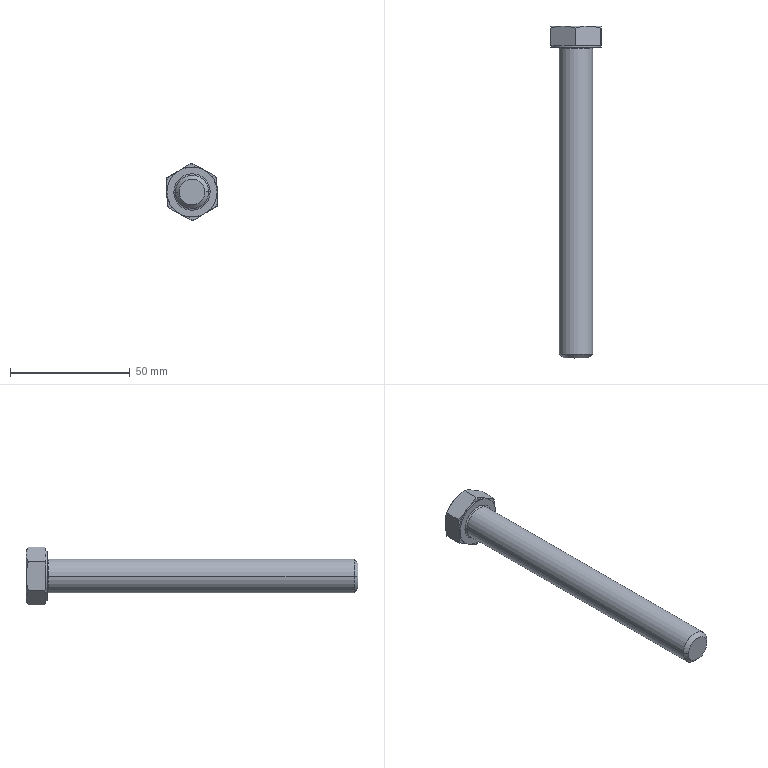Component | SolidWorks | 23HexHeadBolt_GradeAAndB[GBT5782-2000][M14_130_40]-4 | 1 solid | 35 faces | box 21.22 x 138.8 x 24.24 mm | volume 23292 mm3 | plane 15 | cone 14 | cylinder 4 | torus 2 | commonest cylinder face diameters 14 x2 21 x2 | material Steel
STEP:
#1=CARTESIAN_POINT('',(4.247,7.528,24.011));
#2=VERTEX_POINT('',#1);
#3=CARTESIAN_POINT('',(4.799,7.528,24.021));
#4=VERTEX_POINT('',#3);
#5=CARTESIAN_POINT('',(4.523,7.528,24.016));
#6=DIRECTION('',(0.,-1.,0.));
#7=DIRECTION('',(0.9998,0.,0.01816));
#8=AXIS2_PLACEMENT_3D('',#5,#6,#7);
#9=CIRCLE('',#8,0.2756);
#10=EDGE_CURVE('',#2,#4,#9,.T.);
#11=ORIENTED_EDGE('',*,*,#10,.F.);
#12=CARTESIAN_POINT('',(4.224,7.552,24.01));
#13=VERTEX_POINT('',#12);
#14=CARTESIAN_POINT('',(4.224,7.528,24.01));
#15=DIRECTION('',(-0.01816,0.,0.9998));
#16=DIRECTION('',(0.9998,0.,0.01816));
#17=AXIS2_PLACEMENT_3D('',#14,#15,#16);
#18=CIRCLE('',#17,0.02362);
#19=EDGE_CURVE('',#2,#13,#18,.T.);
#20=ORIENTED_EDGE('',*,*,#19,.T.);
#21=CARTESIAN_POINT('',(4.822,7.552,24.021));
#22=VERTEX_POINT('',#21);
#23=CARTESIAN_POINT('',(4.523,7.552,24.016));
#24=DIRECTION('',(0.,1.,0.));
#25=DIRECTION('',(0.9998,0.,0.01816));
#26=AXIS2_PLACEMENT_3D('',#23,#24,#25);
#27=CIRCLE('',#26,0.2992);
#28=EDGE_CURVE('',#22,#13,#27,.T.);
#29=ORIENTED_EDGE('',*,*,#28,.F.);
#30=CARTESIAN_POINT('',(4.822,7.528,24.021));
#31=DIRECTION('',(0.01816,0.,-0.9998));
#32=DIRECTION('',(-0.9998,0.,-0.01816));
#33=AXIS2_PLACEMENT_3D('',#30,#31,#32);
#34=CIRCLE('',#33,0.02362);
#35=EDGE_CURVE('',#4,#22,#34,.T.);
#36=ORIENTED_EDGE('',*,*,#35,.F.);
#37=EDGE_LOOP('',(#11,#20,#29,#36));
#38=FACE_OUTER_BOUND('',#37,.T.);
#39=CARTESIAN_POINT('',(4.523,7.528,24.016));
#40=DIRECTION('',(0.,-1.,0.));
#41=DIRECTION('',(0.9998,0.,0.01816));
#42=AXIS2_PLACEMENT_3D('',#39,#40,#41);
#43=TOROIDAL_SURFACE('',#42,0.2992,0.02362);
#44=ADVANCED_FACE('',(#38),#43,.F.);
#45=CARTESIAN_POINT('',(4.736,2.433,24.02));
#46=VERTEX_POINT('',#45);
#47=CARTESIAN_POINT('',(4.31,2.433,24.012));
#48=VERTEX_POINT('',#47);
#49=CARTESIAN_POINT('',(4.523,2.433,24.016));
#50=DIRECTION('',(0.,-1.,0.));
#51=DIRECTION('',(-0.9998,0.,-0.01816));
#52=AXIS2_PLACEMENT_3D('',#49,#50,#51);
#53=CIRCLE('',#52,0.2126);
#54=EDGE_CURVE('',#46,#48,#53,.T.);
#55=ORIENTED_EDGE('',*,*,#54,.F.);
#56=CARTESIAN_POINT('',(4.799,2.496,24.021));
#57=VERTEX_POINT('',#56);
#58=CARTESIAN_POINT('',(4.799,2.496,24.021));
#59=DIRECTION('',(0.707,0.7071,0.01284));
#60=VECTOR('',#59,39.37);
#61=LINE('',#58,#60);
#62=EDGE_CURVE('',#46,#57,#61,.T.);
#63=ORIENTED_EDGE('',*,*,#62,.T.);
#64=CARTESIAN_POINT('',(4.247,2.496,24.011));
#65=VERTEX_POINT('',#64);
#66=CARTESIAN_POINT('',(4.523,2.496,24.016));
#67=DIRECTION('',(0.,1.,0.));
#68=DIRECTION('',(-0.9998,0.,-0.01816));
#69=AXIS2_PLACEMENT_3D('',#66,#67,#68);
#70=CIRCLE('',#69,0.2756);
#71=EDGE_CURVE('',#65,#57,#70,.T.);
#72=ORIENTED_EDGE('',*,*,#71,.F.);
#73=CARTESIAN_POINT('',(4.247,2.496,24.011));
#74=DIRECTION('',(-0.707,0.7071,-0.01284));
#75=VECTOR('',#74,39.37);
#76=LINE('',#73,#75);
#77=EDGE_CURVE('',#48,#65,#76,.T.);
#78=ORIENTED_EDGE('',*,*,#77,.F.);
#79=EDGE_LOOP('',(#55,#63,#72,#78));
#80=FACE_OUTER_BOUND('',#79,.T.);
#81=CARTESIAN_POINT('',(4.523,2.496,24.016));
#82=DIRECTION('',(0.,1.,0.));
#83=DIRECTION('',(-0.9998,0.,-0.01816));
#84=AXIS2_PLACEMENT_3D('',#81,#82,#83);
#85=CONICAL_SURFACE('',#84,0.2756,0.7854);
#86=ADVANCED_FACE('',(#80),#85,.T.);
#87=ORIENTED_EDGE('',*,*,#71,.T.);
#88=CARTESIAN_POINT('',(4.799,7.898,24.021));
#89=DIRECTION('',(0.,1.,0.));
#90=VECTOR('',#89,39.37);
#91=LINE('',#88,#90);
#92=EDGE_CURVE('',#57,#4,#91,.T.);
#93=ORIENTED_EDGE('',*,*,#92,.T.);
#94=CARTESIAN_POINT('',(4.523,7.528,24.016));
#95=DIRECTION('',(0.,-1.,0.));
#96=DIRECTION('',(0.9998,0.,0.01816));
#97=AXIS2_PLACEMENT_3D('',#94,#95,#96);
#98=CIRCLE('',#97,0.2756);
#99=EDGE_CURVE('',#4,#2,#98,.T.);
#100=ORIENTED_EDGE('',*,*,#99,.T.);
#101=CARTESIAN_POINT('',(4.247,7.898,24.011));
#102=DIRECTION('',(0.,1.,0.));
#103=VECTOR('',#102,39.37);
#104=LINE('',#101,#103);
#105=EDGE_CURVE('',#65,#2,#104,.T.);
#106=ORIENTED_EDGE('',*,*,#105,.F.);
#107=EDGE_LOOP('',(#87,#93,#100,#106));
#108=FACE_OUTER_BOUND('',#107,.T.);
#109=CARTESIAN_POINT('',(4.523,7.898,24.016));
#110=DIRECTION('',(0.,1.,0.));
#111=DIRECTION('',(-0.9998,0.,-0.01816));
#112=AXIS2_PLACEMENT_3D('',#109,#110,#111);
#113=CYLINDRICAL_SURFACE('',#112,0.2756);
#114=ADVANCED_FACE('',(#108),#113,.T.);
#115=CARTESIAN_POINT('',(4.936,7.552,24.023));
#116=VERTEX_POINT('',#115);
#117=CARTESIAN_POINT('',(4.11,7.552,24.008));
#118=VERTEX_POINT('',#117);
#119=CARTESIAN_POINT('',(4.523,7.552,24.016));
#120=DIRECTION('',(0.,-1.,0.));
#121=DIRECTION('',(0.9998,0.,0.01816));
#122=AXIS2_PLACEMENT_3D('',#119,#120,#121);
#123=CIRCLE('',#122,0.4134);
#124=EDGE_CURVE('',#116,#118,#123,.T.);
#125=ORIENTED_EDGE('',*,*,#124,.F.);
#126=CARTESIAN_POINT('',(4.936,7.575,24.023));
#127=VERTEX_POINT('',#126);
#128=CARTESIAN_POINT('',(4.936,7.898,24.023));
#129=DIRECTION('',(0.,1.,0.));
#130=VECTOR('',#129,39.37);
#131=LINE('',#128,#130);
#132=EDGE_CURVE('',#116,#127,#131,.T.);
#133=ORIENTED_EDGE('',*,*,#132,.T.);
#134=CARTESIAN_POINT('',(4.723,7.575,24.377));
#135=VERTEX_POINT('',#134);
#136=CARTESIAN_POINT('',(4.523,7.575,24.016));
#137=DIRECTION('',(0.,1.,0.));
#138=DIRECTION('',(-0.9998,0.,-0.01816));
#139=AXIS2_PLACEMENT_3D('',#136,#137,#138);
#140=CIRCLE('',#139,0.4134);
#141=EDGE_CURVE('',#135,#127,#140,.T.);
#142=ORIENTED_EDGE('',*,*,#141,.F.);
#143=CARTESIAN_POINT('',(4.31,7.575,24.37));
#144=VERTEX_POINT('',#143);
#145=CARTESIAN_POINT('',(4.523,7.575,24.016));
#146=DIRECTION('',(0.,1.,0.));
#147=DIRECTION('',(-0.9998,0.,-0.01816));
#148=AXIS2_PLACEMENT_3D('',#145,#146,#147);
#149=CIRCLE('',#148,0.4134);
#150=EDGE_CURVE('',#144,#135,#149,.T.);
#151=ORIENTED_EDGE('',*,*,#150,.F.);
#152=CARTESIAN_POINT('',(4.11,7.575,24.008));
#153=VERTEX_POINT('',#152);
#154=CARTESIAN_POINT('',(4.523,7.575,24.016));
#155=DIRECTION('',(0.,1.,0.));
#156=DIRECTION('',(-0.9998,0.,-0.01816));
#157=AXIS2_PLACEMENT_3D('',#154,#155,#156);
#158=CIRCLE('',#157,0.4134);
#159=EDGE_CURVE('',#153,#144,#158,.T.);
#160=ORIENTED_EDGE('',*,*,#159,.F.);
#161=CARTESIAN_POINT('',(4.11,7.898,24.008));
#162=DIRECTION('',(0.,1.,0.));
#163=VECTOR('',#162,39.37);
#164=LINE('',#161,#163);
#165=EDGE_CURVE('',#118,#153,#164,.T.);
#166=ORIENTED_EDGE('',*,*,#165,.F.);
#167=EDGE_LOOP('',(#125,#133,#142,#151,#160,#166));
#168=FACE_OUTER_BOUND('',#167,.T.);
#169=CARTESIAN_POINT('',(4.523,7.898,24.016));
#170=DIRECTION('',(0.,1.,0.));
#171=DIRECTION('',(-0.9998,0.,-0.01816));
#172=AXIS2_PLACEMENT_3D('',#169,#170,#171);
#173=CYLINDRICAL_SURFACE('',#172,0.4134);
#174=ADVANCED_FACE('',(#168),#173,.T.);
#175=CARTESIAN_POINT('',(4.888,7.575,24.286));
#176=VERTEX_POINT('',#175);
#177=CARTESIAN_POINT('',(4.932,7.575,24.262));
#178=DIRECTION('',(-0.875,0.,0.4842));
#179=VECTOR('',#178,39.37);
#180=LINE('',#177,#179);
#181=EDGE_CURVE('',#176,#135,#180,.T.);
#182=ORIENTED_EDGE('',*,*,#181,.F.);
#183=CARTESIAN_POINT('',(4.932,7.588,24.262));
#184=VERTEX_POINT('',#183);
#185=CARTESIAN_POINT('',(4.932,7.588,24.262));
#186=CARTESIAN_POINT('',(4.917,7.584,24.27));
#187=CARTESIAN_POINT('',(4.903,7.579,24.278));
#188=CARTESIAN_POINT('',(4.888,7.575,24.286));
#189=B_SPLINE_CURVE_WITH_KNOTS('',3,(#185,#186,#187,#188),.UNSPECIFIED.,.F.,.F.,(4,4),(0.00000024,0.001312),.UNSPECIFIED.);
#190=EDGE_CURVE('',#184,#176,#189,.T.);
#191=ORIENTED_EDGE('',*,*,#190,.F.);
#192=CARTESIAN_POINT('',(4.932,7.861,24.262));
#193=VERTEX_POINT('',#192);
#194=CARTESIAN_POINT('',(4.932,7.552,24.262));
#195=DIRECTION('',(0.,1.,0.));
#196=VECTOR('',#195,39.37);
#197=LINE('',#194,#196);
#198=EDGE_CURVE('',#184,#193,#197,.T.);
#199=ORIENTED_EDGE('',*,*,#198,.T.);
#200=CARTESIAN_POINT('',(4.723,7.898,24.377));
#201=VERTEX_POINT('',#200);
#202=CARTESIAN_POINT('',(4.723,7.898,24.377));
#203=CARTESIAN_POINT('',(4.741,7.898,24.368));
#204=CARTESIAN_POINT('',(4.759,7.897,24.358));
#205=CARTESIAN_POINT('',(4.794,7.894,24.338));
#206=CARTESIAN_POINT('',(4.811,7.891,24.329));
#207=CARTESIAN_POINT('',(4.864,7.882,24.3));
#208=CARTESIAN_POINT('',(4.898,7.872,24.281));
#209=CARTESIAN_POINT('',(4.932,7.861,24.262));
#210=B_SPLINE_CURVE_WITH_KNOTS('',3,(#202,#203,#204,#205,#206,#207,#208,#209),.UNSPECIFIED.,.F.,.F.,(4,2,2,4),(0.006134,0.007662,0.00919,0.01225),.UNSPECIFIED.);
#211=EDGE_CURVE('',#201,#193,#210,.T.);
#212=ORIENTED_EDGE('',*,*,#211,.F.);
#213=CARTESIAN_POINT('',(4.514,7.861,24.493));
#214=VERTEX_POINT('',#213);
#215=CARTESIAN_POINT('',(4.514,7.861,24.493));
#216=CARTESIAN_POINT('',(4.549,7.872,24.474));
#217=CARTESIAN_POINT('',(4.583,7.882,24.455));
#218=CARTESIAN_POINT('',(4.652,7.894,24.417));
#219=CARTESIAN_POINT('',(4.688,7.898,24.397));
#220=CARTESIAN_POINT('',(4.723,7.898,24.377));
#221=B_SPLINE_CURVE_WITH_KNOTS('',3,(#215,#216,#217,#218,#219,#220),.UNSPECIFIED.,.F.,.F.,(4,2,4),(0.00000024,0.003067,0.006134),.UNSPECIFIED.);
#222=EDGE_CURVE('',#214,#201,#221,.T.);
#223=ORIENTED_EDGE('',*,*,#222,.F.);
#224=CARTESIAN_POINT('',(4.514,7.588,24.493));
#225=VERTEX_POINT('',#224);
#226=CARTESIAN_POINT('',(4.514,7.552,24.493));
#227=DIRECTION('',(0.,1.,0.));
#228=VECTOR('',#227,39.37);
#229=LINE('',#226,#228);
#230=EDGE_CURVE('',#225,#214,#229,.T.);
#231=ORIENTED_EDGE('',*,*,#230,.F.);
#232=CARTESIAN_POINT('',(4.558,7.575,24.469));
#233=VERTEX_POINT('',#232);
#234=CARTESIAN_POINT('',(4.558,7.575,24.469));
#235=CARTESIAN_POINT('',(4.544,7.579,24.477));
#236=CARTESIAN_POINT('',(4.529,7.584,24.485));
#237=CARTESIAN_POINT('',(4.514,7.588,24.493));
#238=B_SPLINE_CURVE_WITH_KNOTS('',3,(#234,#235,#236,#237),.UNSPECIFIED.,.F.,.F.,(4,4),(0.01094,0.01225),.UNSPECIFIED.);
#239=EDGE_CURVE('',#233,#225,#238,.T.);
#240=ORIENTED_EDGE('',*,*,#239,.F.);
#241=CARTESIAN_POINT('',(4.932,7.575,24.262));
#242=DIRECTION('',(-0.875,0.,0.4842));
#243=VECTOR('',#242,39.37);
#244=LINE('',#241,#243);
#245=EDGE_CURVE('',#135,#233,#244,.T.);
#246=ORIENTED_EDGE('',*,*,#245,.F.);
#247=EDGE_LOOP('',(#182,#191,#199,#212,#223,#231,#240,#246));
#248=FACE_OUTER_BOUND('',#247,.T.);
#249=CARTESIAN_POINT('',(4.932,7.552,24.262));
#250=DIRECTION('',(-0.4842,0.,-0.875));
#251=DIRECTION('',(0.875,0.,-0.4842));
#252=AXIS2_PLACEMENT_3D('',#249,#250,#251);
#253=PLANE('',#252);
#254=ADVANCED_FACE('',(#248),#253,.F.);
#255=CARTESIAN_POINT('',(4.471,7.575,24.467));
#256=VERTEX_POINT('',#255);
#257=CARTESIAN_POINT('',(4.514,7.575,24.493));
#258=DIRECTION('',(-0.8568,0.,-0.5156));
#259=VECTOR('',#258,39.37);
#260=LINE('',#257,#259);
#261=EDGE_CURVE('',#256,#144,#260,.T.);
#262=ORIENTED_EDGE('',*,*,#261,.F.);
#263=CARTESIAN_POINT('',(4.514,7.588,24.493));
#264=CARTESIAN_POINT('',(4.5,7.584,24.484));
#265=CARTESIAN_POINT('',(4.486,7.579,24.476));
#266=CARTESIAN_POINT('',(4.471,7.575,24.467));
#267=B_SPLINE_CURVE_WITH_KNOTS('',3,(#263,#264,#265,#266),.UNSPECIFIED.,.F.,.F.,(4,4),(0.00000024,0.001312),.UNSPECIFIED.);
#268=EDGE_CURVE('',#225,#256,#267,.T.);
#269=ORIENTED_EDGE('',*,*,#268,.F.);
#270=ORIENTED_EDGE('',*,*,#230,.T.);
#271=CARTESIAN_POINT('',(4.31,7.898,24.37));
#272=VERTEX_POINT('',#271);
#273=CARTESIAN_POINT('',(4.31,7.898,24.37));
#274=CARTESIAN_POINT('',(4.327,7.898,24.38));
#275=CARTESIAN_POINT('',(4.345,7.897,24.391));
#276=CARTESIAN_POINT('',(4.379,7.894,24.412));
#277=CARTESIAN_POINT('',(4.396,7.891,24.422));
#278=CARTESIAN_POINT('',(4.447,7.882,24.453));
#279=CARTESIAN_POINT('',(4.481,7.872,24.473));
#280=CARTESIAN_POINT('',(4.514,7.861,24.493));
#281=B_SPLINE_CURVE_WITH_KNOTS('',3,(#273,#274,#275,#276,#277,#278,#279,#280),.UNSPECIFIED.,.F.,.F.,(4,2,2,4),(0.006134,0.007662,0.00919,0.01225),.UNSPECIFIED.);
#282=EDGE_CURVE('',#272,#214,#281,.T.);
#283=ORIENTED_EDGE('',*,*,#282,.F.);
#284=CARTESIAN_POINT('',(4.105,7.861,24.247));
#285=VERTEX_POINT('',#284);
#286=CARTESIAN_POINT('',(4.105,7.861,24.247));
#287=CARTESIAN_POINT('',(4.139,7.872,24.267));
#288=CARTESIAN_POINT('',(4.173,7.882,24.287));
#289=CARTESIAN_POINT('',(4.241,7.894,24.328));
#290=CARTESIAN_POINT('',(4.275,7.898,24.349));
#291=CARTESIAN_POINT('',(4.31,7.898,24.37));
#292=B_SPLINE_CURVE_WITH_KNOTS('',3,(#286,#287,#288,#289,#290,#291),.UNSPECIFIED.,.F.,.F.,(4,2,4),(0.00000024,0.003067,0.006134),.UNSPECIFIED.);
#293=EDGE_CURVE('',#285,#272,#292,.T.);
#294=ORIENTED_EDGE('',*,*,#293,.F.);
#295=CARTESIAN_POINT('',(4.105,7.588,24.247));
#296=VERTEX_POINT('',#295);
#297=CARTESIAN_POINT('',(4.105,7.552,24.247));
#298=DIRECTION('',(0.,1.,0.));
#299=VECTOR('',#298,39.37);
#300=LINE('',#297,#299);
#301=EDGE_CURVE('',#296,#285,#300,.T.);
#302=ORIENTED_EDGE('',*,*,#301,.F.);
#303=CARTESIAN_POINT('',(4.148,7.575,24.273));
#304=VERTEX_POINT('',#303);
#305=CARTESIAN_POINT('',(4.148,7.575,24.273));
#306=CARTESIAN_POINT('',(4.134,7.579,24.264));
#307=CARTESIAN_POINT('',(4.12,7.584,24.255));
#308=CARTESIAN_POINT('',(4.105,7.588,24.247));
#309=B_SPLINE_CURVE_WITH_KNOTS('',3,(#305,#306,#307,#308),.UNSPECIFIED.,.F.,.F.,(4,4),(0.01094,0.01225),.UNSPECIFIED.);
#310=EDGE_CURVE('',#304,#296,#309,.T.);
#311=ORIENTED_EDGE('',*,*,#310,.F.);
#312=CARTESIAN_POINT('',(4.514,7.575,24.493));
#313=DIRECTION('',(-0.8568,0.,-0.5156));
#314=VECTOR('',#313,39.37);
#315=LINE('',#312,#314);
#316=EDGE_CURVE('',#144,#304,#315,.T.);
#317=ORIENTED_EDGE('',*,*,#316,.F.);
#318=EDGE_LOOP('',(#262,#269,#270,#283,#294,#302,#311,#317));
#319=FACE_OUTER_BOUND('',#318,.T.);
#320=CARTESIAN_POINT('',(4.514,7.552,24.493));
#321=DIRECTION('',(0.5156,0.,-0.8568));
#322=DIRECTION('',(0.8568,0.,0.5156));
#323=AXIS2_PLACEMENT_3D('',#320,#321,#322);
#324=PLANE('',#323);
#325=ADVANCED_FACE('',(#319),#324,.F.);
#326=CARTESIAN_POINT('',(4.106,7.575,24.197));
#327=VERTEX_POINT('',#326);
#328=CARTESIAN_POINT('',(4.105,7.575,24.247));
#329=DIRECTION('',(0.01816,0.,-0.9998));
#330=VECTOR('',#329,39.37);
#331=LINE('',#328,#330);
#332=EDGE_CURVE('',#327,#153,#331,.T.);
#333=ORIENTED_EDGE('',*,*,#332,.F.);
#334=CARTESIAN_POINT('',(4.105,7.588,24.247));
#335=CARTESIAN_POINT('',(4.106,7.584,24.23));
#336=CARTESIAN_POINT('',(4.106,7.579,24.213));
#337=CARTESIAN_POINT('',(4.106,7.575,24.197));
#338=B_SPLINE_CURVE_WITH_KNOTS('',3,(#334,#335,#336,#337),.UNSPECIFIED.,.F.,.F.,(4,4),(0.02875,0.03008),.UNSPECIFIED.);
#339=EDGE_CURVE('',#296,#327,#338,.T.);
#340=ORIENTED_EDGE('',*,*,#339,.F.);
#341=ORIENTED_EDGE('',*,*,#301,.T.);
#342=CARTESIAN_POINT('',(4.11,7.898,24.008));
#343=VERTEX_POINT('',#342);
#344=CARTESIAN_POINT('',(4.11,7.898,24.008));
#345=CARTESIAN_POINT('',(4.109,7.898,24.028));
#346=CARTESIAN_POINT('',(4.109,7.897,24.049));
#347=CARTESIAN_POINT('',(4.108,7.894,24.089));
#348=CARTESIAN_POINT('',(4.108,7.891,24.109));
#349=CARTESIAN_POINT('',(4.107,7.881,24.169));
#350=CARTESIAN_POINT('',(4.106,7.872,24.208));
#351=CARTESIAN_POINT('',(4.105,7.861,24.247));
#352=B_SPLINE_CURVE_WITH_KNOTS('',3,(#344,#345,#346,#347,#348,#349,#350,#351),.UNSPECIFIED.,.F.,.F.,(4,2,2,4),(0.0174,0.01894,0.02047,0.02354),.UNSPECIFIED.);
#353=EDGE_CURVE('',#343,#285,#352,.T.);
#354=ORIENTED_EDGE('',*,*,#353,.F.);
#355=CARTESIAN_POINT('',(4.114,7.861,23.77));
#356=VERTEX_POINT('',#355);
#357=CARTESIAN_POINT('',(4.114,7.861,23.77));
#358=CARTESIAN_POINT('',(4.113,7.872,23.808));
#359=CARTESIAN_POINT('',(4.113,7.882,23.848));
#360=CARTESIAN_POINT('',(4.111,7.895,23.928));
#361=CARTESIAN_POINT('',(4.11,7.898,23.968));
#362=CARTESIAN_POINT('',(4.11,7.898,24.008));
#363=B_SPLINE_CURVE_WITH_KNOTS('',3,(#357,#358,#359,#360,#361,#362),.UNSPECIFIED.,.F.,.F.,(4,2,4),(0.01126,0.01433,0.0174),.UNSPECIFIED.);
#364=EDGE_CURVE('',#356,#343,#363,.T.);
#365=ORIENTED_EDGE('',*,*,#364,.F.);
#366=CARTESIAN_POINT('',(4.114,7.588,23.77));
#367=VERTEX_POINT('',#366);
#368=CARTESIAN_POINT('',(4.114,7.552,23.77));
#369=DIRECTION('',(0.,1.,0.));
#370=VECTOR('',#369,39.37);
#371=LINE('',#368,#370);
#372=EDGE_CURVE('',#367,#356,#371,.T.);
#373=ORIENTED_EDGE('',*,*,#372,.F.);
#374=CARTESIAN_POINT('',(4.113,7.575,23.82));
#375=VERTEX_POINT('',#374);
#376=CARTESIAN_POINT('',(4.113,7.575,23.82));
#377=CARTESIAN_POINT('',(4.113,7.579,23.803));
#378=CARTESIAN_POINT('',(4.114,7.584,23.786));
#379=CARTESIAN_POINT('',(4.114,7.588,23.77));
#380=B_SPLINE_CURVE_WITH_KNOTS('',3,(#376,#377,#378,#379),.UNSPECIFIED.,.F.,.F.,(4,4),(0.03972,0.04103),.UNSPECIFIED.);
#381=EDGE_CURVE('',#375,#367,#380,.T.);
#382=ORIENTED_EDGE('',*,*,#381,.F.);
#383=CARTESIAN_POINT('',(4.105,7.575,24.247));
#384=DIRECTION('',(0.01816,0.,-0.9998));
#385=VECTOR('',#384,39.37);
#386=LINE('',#383,#385);
#387=EDGE_CURVE('',#153,#375,#386,.T.);
#388=ORIENTED_EDGE('',*,*,#387,.F.);
#389=EDGE_LOOP('',(#333,#340,#341,#354,#365,#373,#382,#388));
#390=FACE_OUTER_BOUND('',#389,.T.);
#391=CARTESIAN_POINT('',(4.105,7.552,24.247));
#392=DIRECTION('',(0.9998,0.,0.01816));
#393=DIRECTION('',(0.,1.,0.));
#394=AXIS2_PLACEMENT_3D('',#391,#392,#393);
#395=PLANE('',#394);
#396=ADVANCED_FACE('',(#390),#395,.F.);
#397=CARTESIAN_POINT('',(4.158,7.575,23.745));
#398=VERTEX_POINT('',#397);
#399=CARTESIAN_POINT('',(4.323,7.575,23.654));
#400=VERTEX_POINT('',#399);
#401=CARTESIAN_POINT('',(4.532,7.575,23.538));
#402=DIRECTION('',(0.875,0.,-0.4842));
#403=VECTOR('',#402,39.37);
#404=LINE('',#401,#403);
#405=EDGE_CURVE('',#398,#400,#404,.T.);
#406=ORIENTED_EDGE('',*,*,#405,.F.);
#407=CARTESIAN_POINT('',(4.114,7.588,23.77));
#408=CARTESIAN_POINT('',(4.129,7.584,23.762));
#409=CARTESIAN_POINT('',(4.143,7.579,23.753));
#410=CARTESIAN_POINT('',(4.158,7.575,23.745));
#411=B_SPLINE_CURVE_WITH_KNOTS('',3,(#407,#408,#409,#410),.UNSPECIFIED.,.F.,.F.,(4,4),(0.00000024,0.001312),.UNSPECIFIED.);
#412=EDGE_CURVE('',#367,#398,#411,.T.);
#413=ORIENTED_EDGE('',*,*,#412,.F.);
#414=ORIENTED_EDGE('',*,*,#372,.T.);
#415=CARTESIAN_POINT('',(4.323,7.898,23.654));
#416=VERTEX_POINT('',#415);
#417=CARTESIAN_POINT('',(4.323,7.898,23.654));
#418=CARTESIAN_POINT('',(4.305,7.898,23.664));
#419=CARTESIAN_POINT('',(4.287,7.897,23.674));
#420=CARTESIAN_POINT('',(4.252,7.894,23.693));
#421=CARTESIAN_POINT('',(4.235,7.891,23.703));
#422=CARTESIAN_POINT('',(4.182,7.882,23.732));
#423=CARTESIAN_POINT('',(4.148,7.872,23.751));
#424=CARTESIAN_POINT('',(4.114,7.861,23.77));
#425=B_SPLINE_CURVE_WITH_KNOTS('',3,(#417,#418,#419,#420,#421,#422,#423,#424),.UNSPECIFIED.,.F.,.F.,(4,2,2,4),(0.006134,0.007662,0.00919,0.01225),.UNSPECIFIED.);
#426=EDGE_CURVE('',#416,#356,#425,.T.);
#427=ORIENTED_EDGE('',*,*,#426,.F.);
#428=CARTESIAN_POINT('',(4.532,7.861,23.538));
#429=VERTEX_POINT('',#428);
#430=CARTESIAN_POINT('',(4.532,7.861,23.538));
#431=CARTESIAN_POINT('',(4.498,7.872,23.557));
#432=CARTESIAN_POINT('',(4.463,7.882,23.576));
#433=CARTESIAN_POINT('',(4.394,7.894,23.615));
#434=CARTESIAN_POINT('',(4.358,7.898,23.634));
#435=CARTESIAN_POINT('',(4.323,7.898,23.654));
#436=B_SPLINE_CURVE_WITH_KNOTS('',3,(#430,#431,#432,#433,#434,#435),.UNSPECIFIED.,.F.,.F.,(4,2,4),(0.00000024,0.003067,0.006134),.UNSPECIFIED.);
#437=EDGE_CURVE('',#429,#416,#436,.T.);
#438=ORIENTED_EDGE('',*,*,#437,.F.);
#439=CARTESIAN_POINT('',(4.532,7.588,23.538));
#440=VERTEX_POINT('',#439);
#441=CARTESIAN_POINT('',(4.532,7.552,23.538));
#442=DIRECTION('',(0.,1.,0.));
#443=VECTOR('',#442,39.37);
#444=LINE('',#441,#443);
#445=EDGE_CURVE('',#440,#429,#444,.T.);
#446=ORIENTED_EDGE('',*,*,#445,.F.);
#447=CARTESIAN_POINT('',(4.488,7.575,23.563));
#448=VERTEX_POINT('',#447);
#449=CARTESIAN_POINT('',(4.488,7.575,23.563));
#450=CARTESIAN_POINT('',(4.502,7.579,23.555));
#451=CARTESIAN_POINT('',(4.517,7.584,23.547));
#452=CARTESIAN_POINT('',(4.532,7.588,23.538));
#453=B_SPLINE_CURVE_WITH_KNOTS('',3,(#449,#450,#451,#452),.UNSPECIFIED.,.F.,.F.,(4,4),(0.01094,0.01225),.UNSPECIFIED.);
#454=EDGE_CURVE('',#448,#440,#453,.T.);
#455=ORIENTED_EDGE('',*,*,#454,.F.);
#456=CARTESIAN_POINT('',(4.532,7.575,23.538));
#457=DIRECTION('',(0.875,0.,-0.4842));
#458=VECTOR('',#457,39.37);
#459=LINE('',#456,#458);
#460=EDGE_CURVE('',#400,#448,#459,.T.);
#461=ORIENTED_EDGE('',*,*,#460,.F.);
#462=EDGE_LOOP('',(#406,#413,#414,#427,#438,#446,#455,#461));
#463=FACE_OUTER_BOUND('',#462,.T.);
#464=CARTESIAN_POINT('',(4.532,7.552,23.538));
#465=DIRECTION('',(0.4842,0.,0.875));
#466=DIRECTION('',(-0.875,0.,0.4842));
#467=AXIS2_PLACEMENT_3D('',#464,#465,#466);
#468=PLANE('',#467);
#469=ADVANCED_FACE('',(#463),#468,.F.);
#470=CARTESIAN_POINT('',(4.575,7.575,23.564));
#471=VERTEX_POINT('',#470);
#472=CARTESIAN_POINT('',(4.736,7.575,23.662));
#473=VERTEX_POINT('',#472);
#474=CARTESIAN_POINT('',(4.941,7.575,23.785));
#475=DIRECTION('',(0.8568,0.,0.5156));
#476=VECTOR('',#475,39.37);
#477=LINE('',#474,#476);
#478=EDGE_CURVE('',#471,#473,#477,.T.);
#479=ORIENTED_EDGE('',*,*,#478,.F.);
#480=CARTESIAN_POINT('',(4.532,7.588,23.538));
#481=CARTESIAN_POINT('',(4.546,7.584,23.547));
#482=CARTESIAN_POINT('',(4.56,7.579,23.556));
#483=CARTESIAN_POINT('',(4.575,7.575,23.564));
#484=B_SPLINE_CURVE_WITH_KNOTS('',3,(#480,#481,#482,#483),.UNSPECIFIED.,.F.,.F.,(4,4),(0.00000024,0.001312),.UNSPECIFIED.);
#485=EDGE_CURVE('',#440,#471,#484,.T.);
#486=ORIENTED_EDGE('',*,*,#485,.F.);
#487=ORIENTED_EDGE('',*,*,#445,.T.);
#488=CARTESIAN_POINT('',(4.736,7.898,23.662));
#489=VERTEX_POINT('',#488);
#490=CARTESIAN_POINT('',(4.736,7.898,23.662));
#491=CARTESIAN_POINT('',(4.719,7.898,23.651));
#492=CARTESIAN_POINT('',(4.701,7.897,23.641));
#493=CARTESIAN_POINT('',(4.667,7.894,23.62));
#494=CARTESIAN_POINT('',(4.65,7.891,23.61));
#495=CARTESIAN_POINT('',(4.599,7.882,23.579));
#496=CARTESIAN_POINT('',(4.565,7.872,23.559));
#497=CARTESIAN_POINT('',(4.532,7.861,23.538));
#498=B_SPLINE_CURVE_WITH_KNOTS('',3,(#490,#491,#492,#493,#494,#495,#496,#497),.UNSPECIFIED.,.F.,.F.,(4,2,2,4),(0.006134,0.007662,0.00919,0.01225),.UNSPECIFIED.);
#499=EDGE_CURVE('',#489,#429,#498,.T.);
#500=ORIENTED_EDGE('',*,*,#499,.F.);
#501=CARTESIAN_POINT('',(4.941,7.861,23.785));
#502=VERTEX_POINT('',#501);
#503=CARTESIAN_POINT('',(4.941,7.861,23.785));
#504=CARTESIAN_POINT('',(4.907,7.872,23.764));
#505=CARTESIAN_POINT('',(4.874,7.882,23.744));
#506=CARTESIAN_POINT('',(4.805,7.894,23.703));
#507=CARTESIAN_POINT('',(4.771,7.898,23.683));
#508=CARTESIAN_POINT('',(4.736,7.898,23.662));
#509=B_SPLINE_CURVE_WITH_KNOTS('',3,(#503,#504,#505,#506,#507,#508),.UNSPECIFIED.,.F.,.F.,(4,2,4),(0.00000024,0.003067,0.006134),.UNSPECIFIED.);
#510=EDGE_CURVE('',#502,#489,#509,.T.);
#511=ORIENTED_EDGE('',*,*,#510,.F.);
#512=CARTESIAN_POINT('',(4.941,7.588,23.785));
#513=VERTEX_POINT('',#512);
#514=CARTESIAN_POINT('',(4.941,7.552,23.785));
#515=DIRECTION('',(0.,1.,0.));
#516=VECTOR('',#515,39.37);
#517=LINE('',#514,#516);
#518=EDGE_CURVE('',#513,#502,#517,.T.);
#519=ORIENTED_EDGE('',*,*,#518,.F.);
#520=CARTESIAN_POINT('',(4.898,7.575,23.759));
#521=VERTEX_POINT('',#520);
#522=CARTESIAN_POINT('',(4.898,7.575,23.759));
#523=CARTESIAN_POINT('',(4.912,7.579,23.767));
#524=CARTESIAN_POINT('',(4.926,7.584,23.776));
#525=CARTESIAN_POINT('',(4.941,7.588,23.785));
#526=B_SPLINE_CURVE_WITH_KNOTS('',3,(#522,#523,#524,#525),.UNSPECIFIED.,.F.,.F.,(4,4),(0.01094,0.01225),.UNSPECIFIED.);
#527=EDGE_CURVE('',#521,#513,#526,.T.);
#528=ORIENTED_EDGE('',*,*,#527,.F.);
#529=CARTESIAN_POINT('',(4.941,7.575,23.785));
#530=DIRECTION('',(0.8568,0.,0.5156));
#531=VECTOR('',#530,39.37);
#532=LINE('',#529,#531);
#533=EDGE_CURVE('',#473,#521,#532,.T.);
#534=ORIENTED_EDGE('',*,*,#533,.F.);
#535=EDGE_LOOP('',(#479,#486,#487,#500,#511,#519,#528,#534));
#536=FACE_OUTER_BOUND('',#535,.T.);
#537=CARTESIAN_POINT('',(4.941,7.552,23.785));
#538=DIRECTION('',(-0.5156,0.,0.8568));
#539=DIRECTION('',(-0.8568,0.,-0.5156));
#540=AXIS2_PLACEMENT_3D('',#537,#538,#539);
#541=PLANE('',#540);
#542=ADVANCED_FACE('',(#536),#541,.F.);
#543=CARTESIAN_POINT('',(4.94,7.575,23.835));
#544=VERTEX_POINT('',#543);
#545=CARTESIAN_POINT('',(4.932,7.575,24.262));
#546=DIRECTION('',(-0.01816,0.,0.9998));
#547=VECTOR('',#546,39.37);
#548=LINE('',#545,#547);
#549=EDGE_CURVE('',#544,#127,#548,.T.);
#550=ORIENTED_EDGE('',*,*,#549,.F.);
#551=CARTESIAN_POINT('',(4.941,7.588,23.785));
#552=CARTESIAN_POINT('',(4.94,7.584,23.801));
#553=CARTESIAN_POINT('',(4.94,7.579,23.818));
#554=CARTESIAN_POINT('',(4.94,7.575,23.835));
#555=B_SPLINE_CURVE_WITH_KNOTS('',3,(#551,#552,#553,#554),.UNSPECIFIED.,.F.,.F.,(4,4),(0.01126,0.01258),.UNSPECIFIED.);
#556=EDGE_CURVE('',#513,#544,#555,.T.);
#557=ORIENTED_EDGE('',*,*,#556,.F.);
#558=ORIENTED_EDGE('',*,*,#518,.T.);
#559=CARTESIAN_POINT('',(4.936,7.898,24.023));
#560=VERTEX_POINT('',#559);
#561=CARTESIAN_POINT('',(4.936,7.898,24.023));
#562=CARTESIAN_POINT('',(4.937,7.898,23.983));
#563=CARTESIAN_POINT('',(4.938,7.895,23.943));
#564=CARTESIAN_POINT('',(4.939,7.882,23.863));
#565=CARTESIAN_POINT('',(4.94,7.872,23.823));
#566=CARTESIAN_POINT('',(4.941,7.861,23.785));
#567=B_SPLINE_CURVE_WITH_KNOTS('',3,(#561,#562,#563,#564,#565,#566),.UNSPECIFIED.,.F.,.F.,(4,2,4),(0.03489,0.03796,0.04103),.UNSPECIFIED.);
#568=EDGE_CURVE('',#560,#502,#567,.T.);
#569=ORIENTED_EDGE('',*,*,#568,.F.);
#570=CARTESIAN_POINT('',(4.932,7.861,24.262));
#571=CARTESIAN_POINT('',(4.933,7.872,24.223));
#572=CARTESIAN_POINT('',(4.933,7.881,24.184));
#573=CARTESIAN_POINT('',(4.934,7.891,24.124));
#574=CARTESIAN_POINT('',(4.935,7.894,24.104));
#575=CARTESIAN_POINT('',(4.936,7.897,24.064));
#576=CARTESIAN_POINT('',(4.936,7.898,24.043));
#577=CARTESIAN_POINT('',(4.936,7.898,24.023));
#578=B_SPLINE_CURVE_WITH_KNOTS('',3,(#570,#571,#572,#573,#574,#575,#576,#577),.UNSPECIFIED.,.F.,.F.,(4,2,2,4),(0.02875,0.03182,0.03336,0.03489),.UNSPECIFIED.);
#579=EDGE_CURVE('',#193,#560,#578,.T.);
#580=ORIENTED_EDGE('',*,*,#579,.F.);
#581=ORIENTED_EDGE('',*,*,#198,.F.);
#582=CARTESIAN_POINT('',(4.933,7.575,24.212));
#583=VERTEX_POINT('',#582);
#584=CARTESIAN_POINT('',(4.933,7.575,24.212));
#585=CARTESIAN_POINT('',(4.933,7.579,24.228));
#586=CARTESIAN_POINT('',(4.932,7.584,24.245));
#587=CARTESIAN_POINT('',(4.932,7.588,24.262));
#588=B_SPLINE_CURVE_WITH_KNOTS('',3,(#584,#585,#586,#587),.UNSPECIFIED.,.F.,.F.,(4,4),(0.02222,0.02354),.UNSPECIFIED.);
#589=EDGE_CURVE('',#583,#184,#588,.T.);
#590=ORIENTED_EDGE('',*,*,#589,.F.);
#591=CARTESIAN_POINT('',(4.932,7.575,24.262));
#592=DIRECTION('',(-0.01816,0.,0.9998));
#593=VECTOR('',#592,39.37);
#594=LINE('',#591,#593);
#595=EDGE_CURVE('',#127,#583,#594,.T.);
#596=ORIENTED_EDGE('',*,*,#595,.F.);
#597=EDGE_LOOP('',(#550,#557,#558,#569,#580,#581,#590,#596));
#598=FACE_OUTER_BOUND('',#597,.T.);
#599=CARTESIAN_POINT('',(4.932,7.552,24.262));
#600=DIRECTION('',(-0.9998,0.,-0.01816));
#601=DIRECTION('',(0.,-1.,0.));
#602=AXIS2_PLACEMENT_3D('',#599,#600,#601);
#603=PLANE('',#602);
#604=ADVANCED_FACE('',(#598),#603,.F.);
#605=ORIENTED_EDGE('',*,*,#556,.T.);
#606=CARTESIAN_POINT('',(4.523,7.575,24.016));
#607=DIRECTION('',(0.,1.,0.));
#608=DIRECTION('',(0.9998,0.,0.01816));
#609=AXIS2_PLACEMENT_3D('',#606,#607,#608);
#610=CIRCLE('',#609,0.4543);
#611=EDGE_CURVE('',#544,#521,#610,.T.);
#612=ORIENTED_EDGE('',*,*,#611,.T.);
#613=ORIENTED_EDGE('',*,*,#527,.T.);
#614=EDGE_LOOP('',(#605,#612,#613));
#615=FACE_OUTER_BOUND('',#614,.T.);
#616=CARTESIAN_POINT('',(4.523,7.702,24.016));
#617=DIRECTION('',(0.,1.,0.));
#618=DIRECTION('',(-0.9998,0.,-0.01816));
#619=AXIS2_PLACEMENT_3D('',#616,#617,#618);
#620=CONICAL_SURFACE('',#619,0.6742,1.047);
#621=ADVANCED_FACE('',(#615),#620,.T.);
#622=ORIENTED_EDGE('',*,*,#485,.T.);
#623=CARTESIAN_POINT('',(4.523,7.575,24.016));
#624=DIRECTION('',(0.,1.,0.));
#625=DIRECTION('',(0.9998,0.,0.01816));
#626=AXIS2_PLACEMENT_3D('',#623,#624,#625);
#627=CIRCLE('',#626,0.4543);
#628=EDGE_CURVE('',#471,#448,#627,.T.);
#629=ORIENTED_EDGE('',*,*,#628,.T.);
#630=ORIENTED_EDGE('',*,*,#454,.T.);
#631=EDGE_LOOP('',(#622,#629,#630));
#632=FACE_OUTER_BOUND('',#631,.T.);
#633=CARTESIAN_POINT('',(4.523,7.702,24.016));
#634=DIRECTION('',(0.,1.,0.));
#635=DIRECTION('',(-0.9998,0.,-0.01816));
#636=AXIS2_PLACEMENT_3D('',#633,#634,#635);
#637=CONICAL_SURFACE('',#636,0.6742,1.047);
#638=ADVANCED_FACE('',(#632),#637,.T.);
#639=ORIENTED_EDGE('',*,*,#412,.T.);
#640=CARTESIAN_POINT('',(4.523,7.575,24.016));
#641=DIRECTION('',(0.,1.,0.));
#642=DIRECTION('',(0.9998,0.,0.01816));
#643=AXIS2_PLACEMENT_3D('',#640,#641,#642);
#644=CIRCLE('',#643,0.4543);
#645=EDGE_CURVE('',#398,#375,#644,.T.);
#646=ORIENTED_EDGE('',*,*,#645,.T.);
#647=ORIENTED_EDGE('',*,*,#381,.T.);
#648=EDGE_LOOP('',(#639,#646,#647));
#649=FACE_OUTER_BOUND('',#648,.T.);
#650=CARTESIAN_POINT('',(4.523,7.702,24.016));
#651=DIRECTION('',(0.,1.,0.));
#652=DIRECTION('',(-0.9998,0.,-0.01816));
#653=AXIS2_PLACEMENT_3D('',#650,#651,#652);
#654=CONICAL_SURFACE('',#653,0.6742,1.047);
#655=ADVANCED_FACE('',(#649),#654,.T.);
#656=ORIENTED_EDGE('',*,*,#339,.T.);
#657=CARTESIAN_POINT('',(4.523,7.575,24.016));
#658=DIRECTION('',(0.,1.,0.));
#659=DIRECTION('',(0.9998,0.,0.01816));
#660=AXIS2_PLACEMENT_3D('',#657,#658,#659);
#661=CIRCLE('',#660,0.4543);
#662=EDGE_CURVE('',#327,#304,#661,.T.);
#663=ORIENTED_EDGE('',*,*,#662,.T.);
#664=ORIENTED_EDGE('',*,*,#310,.T.);
#665=EDGE_LOOP('',(#656,#663,#664));
#666=FACE_OUTER_BOUND('',#665,.T.);
#667=CARTESIAN_POINT('',(4.523,7.702,24.016));
#668=DIRECTION('',(0.,1.,0.));
#669=DIRECTION('',(-0.9998,0.,-0.01816));
#670=AXIS2_PLACEMENT_3D('',#667,#668,#669);
#671=CONICAL_SURFACE('',#670,0.6742,1.047);
#672=ADVANCED_FACE('',(#666),#671,.T.);
#673=ORIENTED_EDGE('',*,*,#268,.T.);
#674=CARTESIAN_POINT('',(4.523,7.575,24.016));
#675=DIRECTION('',(0.,1.,0.));
#676=DIRECTION('',(0.9998,0.,0.01816));
#677=AXIS2_PLACEMENT_3D('',#674,#675,#676);
#678=CIRCLE('',#677,0.4543);
#679=EDGE_CURVE('',#256,#233,#678,.T.);
#680=ORIENTED_EDGE('',*,*,#679,.T.);
#681=ORIENTED_EDGE('',*,*,#239,.T.);
#682=EDGE_LOOP('',(#673,#680,#681));
#683=FACE_OUTER_BOUND('',#682,.T.);
#684=CARTESIAN_POINT('',(4.523,7.702,24.016));
#685=DIRECTION('',(0.,1.,0.));
#686=DIRECTION('',(-0.9998,0.,-0.01816));
#687=AXIS2_PLACEMENT_3D('',#684,#685,#686);
#688=CONICAL_SURFACE('',#687,0.6742,1.047);
#689=ADVANCED_FACE('',(#683),#688,.T.);
#690=ORIENTED_EDGE('',*,*,#190,.T.);
#691=CARTESIAN_POINT('',(4.523,7.575,24.016));
#692=DIRECTION('',(0.,1.,0.));
#693=DIRECTION('',(0.9998,0.,0.01816));
#694=AXIS2_PLACEMENT_3D('',#691,#692,#693);
#695=CIRCLE('',#694,0.4543);
#696=EDGE_CURVE('',#176,#583,#695,.T.);
#697=ORIENTED_EDGE('',*,*,#696,.T.);
#698=ORIENTED_EDGE('',*,*,#589,.T.);
#699=EDGE_LOOP('',(#690,#697,#698));
#700=FACE_OUTER_BOUND('',#699,.T.);
#701=CARTESIAN_POINT('',(4.523,7.702,24.016));
#702=DIRECTION('',(0.,1.,0.));
#703=DIRECTION('',(-0.9998,0.,-0.01816));
#704=AXIS2_PLACEMENT_3D('',#701,#702,#703);
#705=CONICAL_SURFACE('',#704,0.6742,1.047);
#706=ADVANCED_FACE('',(#700),#705,.T.);
#707=ORIENTED_EDGE('',*,*,#510,.T.);
#708=CARTESIAN_POINT('',(4.523,7.898,24.016));
#709=DIRECTION('',(0.,-1.,0.));
#710=DIRECTION('',(0.9998,0.,0.01816));
#711=AXIS2_PLACEMENT_3D('',#708,#709,#710);
#712=CIRCLE('',#711,0.4134);
#713=EDGE_CURVE('',#489,#560,#712,.T.);
#714=ORIENTED_EDGE('',*,*,#713,.T.);
#715=ORIENTED_EDGE('',*,*,#568,.T.);
#716=EDGE_LOOP('',(#707,#714,#715));
#717=FACE_OUTER_BOUND('',#716,.T.);
#718=CARTESIAN_POINT('',(4.523,7.898,24.016));
#719=DIRECTION('',(0.,-1.,0.));
#720=DIRECTION('',(0.9998,0.,0.01816));
#721=AXIS2_PLACEMENT_3D('',#718,#719,#720);
#722=CONICAL_SURFACE('',#721,0.4134,1.047);
#723=ADVANCED_FACE('',(#717),#722,.T.);
#724=ORIENTED_EDGE('',*,*,#437,.T.);
#725=CARTESIAN_POINT('',(4.523,7.898,24.016));
#726=DIRECTION('',(0.,-1.,0.));
#727=DIRECTION('',(0.9998,0.,0.01816));
#728=AXIS2_PLACEMENT_3D('',#725,#726,#727);
#729=CIRCLE('',#728,0.4134);
#730=EDGE_CURVE('',#416,#489,#729,.T.);
#731=ORIENTED_EDGE('',*,*,#730,.T.);
#732=ORIENTED_EDGE('',*,*,#499,.T.);
#733=EDGE_LOOP('',(#724,#731,#732));
#734=FACE_OUTER_BOUND('',#733,.T.);
#735=CARTESIAN_POINT('',(4.523,7.898,24.016));
#736=DIRECTION('',(0.,-1.,0.));
#737=DIRECTION('',(0.9998,0.,0.01816));
#738=AXIS2_PLACEMENT_3D('',#735,#736,#737);
#739=CONICAL_SURFACE('',#738,0.4134,1.047);
#740=ADVANCED_FACE('',(#734),#739,.T.);
#741=ORIENTED_EDGE('',*,*,#364,.T.);
#742=CARTESIAN_POINT('',(4.523,7.898,24.016));
#743=DIRECTION('',(0.,-1.,0.));
#744=DIRECTION('',(0.9998,0.,0.01816));
#745=AXIS2_PLACEMENT_3D('',#742,#743,#744);
#746=CIRCLE('',#745,0.4134);
#747=EDGE_CURVE('',#343,#416,#746,.T.);
#748=ORIENTED_EDGE('',*,*,#747,.T.);
#749=ORIENTED_EDGE('',*,*,#426,.T.);
#750=EDGE_LOOP('',(#741,#748,#749));
#751=FACE_OUTER_BOUND('',#750,.T.);
#752=CARTESIAN_POINT('',(4.523,7.898,24.016));
#753=DIRECTION('',(0.,-1.,0.));
#754=DIRECTION('',(0.9998,0.,0.01816));
#755=AXIS2_PLACEMENT_3D('',#752,#753,#754);
#756=CONICAL_SURFACE('',#755,0.4134,1.047);
#757=ADVANCED_FACE('',(#751),#756,.T.);
#758=ORIENTED_EDGE('',*,*,#353,.T.);
#759=ORIENTED_EDGE('',*,*,#293,.T.);
#760=CARTESIAN_POINT('',(4.523,7.898,24.016));
#761=DIRECTION('',(0.,1.,0.));
#762=DIRECTION('',(-0.9998,0.,-0.01816));
#763=AXIS2_PLACEMENT_3D('',#760,#761,#762);
#764=CIRCLE('',#763,0.4134);
#765=EDGE_CURVE('',#343,#272,#764,.T.);
#766=ORIENTED_EDGE('',*,*,#765,.F.);
#767=EDGE_LOOP('',(#758,#759,#766));
#768=FACE_OUTER_BOUND('',#767,.T.);
#769=CARTESIAN_POINT('',(4.523,7.898,24.016));
#770=DIRECTION('',(0.,-1.,0.));
#771=DIRECTION('',(0.9998,0.,0.01816));
#772=AXIS2_PLACEMENT_3D('',#769,#770,#771);
#773=CONICAL_SURFACE('',#772,0.4134,1.047);
#774=ADVANCED_FACE('',(#768),#773,.T.);
#775=ORIENTED_EDGE('',*,*,#282,.T.);
#776=ORIENTED_EDGE('',*,*,#222,.T.);
#777=CARTESIAN_POINT('',(4.523,7.898,24.016));
#778=DIRECTION('',(0.,-1.,0.));
#779=DIRECTION('',(0.9998,0.,0.01816));
#780=AXIS2_PLACEMENT_3D('',#777,#778,#779);
#781=CIRCLE('',#780,0.4134);
#782=EDGE_CURVE('',#201,#272,#781,.T.);
#783=ORIENTED_EDGE('',*,*,#782,.T.);
#784=EDGE_LOOP('',(#775,#776,#783));
#785=FACE_OUTER_BOUND('',#784,.T.);
#786=CARTESIAN_POINT('',(4.523,7.898,24.016));
#787=DIRECTION('',(0.,-1.,0.));
#788=DIRECTION('',(0.9998,0.,0.01816));
#789=AXIS2_PLACEMENT_3D('',#786,#787,#788);
#790=CONICAL_SURFACE('',#789,0.4134,1.047);
#791=ADVANCED_FACE('',(#785),#790,.T.);
#792=ORIENTED_EDGE('',*,*,#211,.T.);
#793=ORIENTED_EDGE('',*,*,#579,.T.);
#794=CARTESIAN_POINT('',(4.523,7.898,24.016));
#795=DIRECTION('',(0.,-1.,0.));
#796=DIRECTION('',(0.9998,0.,0.01816));
#797=AXIS2_PLACEMENT_3D('',#794,#795,#796);
#798=CIRCLE('',#797,0.4134);
#799=EDGE_CURVE('',#560,#201,#798,.T.);
#800=ORIENTED_EDGE('',*,*,#799,.T.);
#801=EDGE_LOOP('',(#792,#793,#800));
#802=FACE_OUTER_BOUND('',#801,.T.);
#803=CARTESIAN_POINT('',(4.523,7.898,24.016));
#804=DIRECTION('',(0.,-1.,0.));
#805=DIRECTION('',(0.9998,0.,0.01816));
#806=AXIS2_PLACEMENT_3D('',#803,#804,#805);
#807=CONICAL_SURFACE('',#806,0.4134,1.047);
#808=ADVANCED_FACE('',(#802),#807,.T.);
#809=ORIENTED_EDGE('',*,*,#799,.F.);
#810=ORIENTED_EDGE('',*,*,#713,.F.);
#811=ORIENTED_EDGE('',*,*,#730,.F.);
#812=ORIENTED_EDGE('',*,*,#747,.F.);
#813=ORIENTED_EDGE('',*,*,#765,.T.);
#814=ORIENTED_EDGE('',*,*,#782,.F.);
#815=EDGE_LOOP('',(#809,#810,#811,#812,#813,#814));
#816=FACE_OUTER_BOUND('',#815,.T.);
#817=CARTESIAN_POINT('',(4.514,7.898,24.493));
#818=DIRECTION('',(0.,-1.,0.));
#819=DIRECTION('',(0.9998,0.,0.01816));
#820=AXIS2_PLACEMENT_3D('',#817,#818,#819);
#821=PLANE('',#820);
#822=ADVANCED_FACE('',(#816),#821,.F.);
#823=ORIENTED_EDGE('',*,*,#387,.T.);
#824=ORIENTED_EDGE('',*,*,#645,.F.);
#825=ORIENTED_EDGE('',*,*,#405,.T.);
#826=CARTESIAN_POINT('',(4.523,7.575,24.016));
#827=DIRECTION('',(0.,1.,0.));
#828=DIRECTION('',(-0.9998,0.,-0.01816));
#829=AXIS2_PLACEMENT_3D('',#826,#827,#828);
#830=CIRCLE('',#829,0.4134);
#831=EDGE_CURVE('',#400,#153,#830,.T.);
#832=ORIENTED_EDGE('',*,*,#831,.T.);
#833=EDGE_LOOP('',(#823,#824,#825,#832));
#834=FACE_OUTER_BOUND('',#833,.T.);
#835=CARTESIAN_POINT('',(4.516,7.575,24.429));
#836=DIRECTION('',(0.,-1.,0.));
#837=DIRECTION('',(0.9998,0.,0.01816));
#838=AXIS2_PLACEMENT_3D('',#835,#836,#837);
#839=PLANE('',#838);
#840=ADVANCED_FACE('',(#834),#839,.T.);
#841=ORIENTED_EDGE('',*,*,#261,.T.);
#842=ORIENTED_EDGE('',*,*,#150,.T.);
#843=ORIENTED_EDGE('',*,*,#245,.T.);
#844=ORIENTED_EDGE('',*,*,#679,.F.);
#845=EDGE_LOOP('',(#841,#842,#843,#844));
#846=FACE_OUTER_BOUND('',#845,.T.);
#847=CARTESIAN_POINT('',(4.516,7.575,24.429));
#848=DIRECTION('',(0.,-1.,0.));
#849=DIRECTION('',(0.9998,0.,0.01816));
#850=AXIS2_PLACEMENT_3D('',#847,#848,#849);
#851=PLANE('',#850);
#852=ADVANCED_FACE('',(#846),#851,.T.);
#853=ORIENTED_EDGE('',*,*,#460,.T.);
#854=ORIENTED_EDGE('',*,*,#628,.F.);
#855=ORIENTED_EDGE('',*,*,#478,.T.);
#856=CARTESIAN_POINT('',(4.523,7.575,24.016));
#857=DIRECTION('',(0.,1.,0.));
#858=DIRECTION('',(-0.9998,0.,-0.01816));
#859=AXIS2_PLACEMENT_3D('',#856,#857,#858);
#860=CIRCLE('',#859,0.4134);
#861=EDGE_CURVE('',#473,#400,#860,.T.);
#862=ORIENTED_EDGE('',*,*,#861,.T.);
#863=EDGE_LOOP('',(#853,#854,#855,#862));
#864=FACE_OUTER_BOUND('',#863,.T.);
#865=CARTESIAN_POINT('',(4.516,7.575,24.429));
#866=DIRECTION('',(0.,-1.,0.));
#867=DIRECTION('',(0.9998,0.,0.01816));
#868=AXIS2_PLACEMENT_3D('',#865,#866,#867);
#869=PLANE('',#868);
#870=ADVANCED_FACE('',(#864),#869,.T.);
#871=ORIENTED_EDGE('',*,*,#533,.T.);
#872=ORIENTED_EDGE('',*,*,#611,.F.);
#873=ORIENTED_EDGE('',*,*,#549,.T.);
#874=CARTESIAN_POINT('',(4.523,7.575,24.016));
#875=DIRECTION('',(0.,1.,0.));
#876=DIRECTION('',(-0.9998,0.,-0.01816));
#877=AXIS2_PLACEMENT_3D('',#874,#875,#876);
#878=CIRCLE('',#877,0.4134);
#879=EDGE_CURVE('',#127,#473,#878,.T.);
#880=ORIENTED_EDGE('',*,*,#879,.T.);
#881=EDGE_LOOP('',(#871,#872,#873,#880));
#882=FACE_OUTER_BOUND('',#881,.T.);
#883=CARTESIAN_POINT('',(4.516,7.575,24.429));
#884=DIRECTION('',(0.,-1.,0.));
#885=DIRECTION('',(0.9998,0.,0.01816));
#886=AXIS2_PLACEMENT_3D('',#883,#884,#885);
#887=PLANE('',#886);
#888=ADVANCED_FACE('',(#882),#887,.T.);
#889=ORIENTED_EDGE('',*,*,#181,.T.);
#890=ORIENTED_EDGE('',*,*,#141,.T.);
#891=ORIENTED_EDGE('',*,*,#595,.T.);
#892=ORIENTED_EDGE('',*,*,#696,.F.);
#893=EDGE_LOOP('',(#889,#890,#891,#892));
#894=FACE_OUTER_BOUND('',#893,.T.);
#895=CARTESIAN_POINT('',(4.516,7.575,24.429));
#896=DIRECTION('',(0.,-1.,0.));
#897=DIRECTION('',(0.9998,0.,0.01816));
#898=AXIS2_PLACEMENT_3D('',#895,#896,#897);
#899=PLANE('',#898);
#900=ADVANCED_FACE('',(#894),#899,.T.);
#901=ORIENTED_EDGE('',*,*,#132,.F.);
#902=CARTESIAN_POINT('',(4.523,7.552,24.016));
#903=DIRECTION('',(0.,-1.,0.));
#904=DIRECTION('',(0.9998,0.,0.01816));
#905=AXIS2_PLACEMENT_3D('',#902,#903,#904);
#906=CIRCLE('',#905,0.4134);
#907=EDGE_CURVE('',#118,#116,#906,.T.);
#908=ORIENTED_EDGE('',*,*,#907,.F.);
#909=ORIENTED_EDGE('',*,*,#165,.T.);
#910=ORIENTED_EDGE('',*,*,#831,.F.);
#911=ORIENTED_EDGE('',*,*,#861,.F.);
#912=ORIENTED_EDGE('',*,*,#879,.F.);
#913=EDGE_LOOP('',(#901,#908,#909,#910,#911,#912));
#914=FACE_OUTER_BOUND('',#913,.T.);
#915=CARTESIAN_POINT('',(4.523,7.898,24.016));
#916=DIRECTION('',(0.,1.,0.));
#917=DIRECTION('',(-0.9998,0.,-0.01816));
#918=AXIS2_PLACEMENT_3D('',#915,#916,#917);
#919=CYLINDRICAL_SURFACE('',#918,0.4134);
#920=ADVANCED_FACE('',(#914),#919,.T.);
#921=ORIENTED_EDGE('',*,*,#332,.T.);
#922=ORIENTED_EDGE('',*,*,#159,.T.);
#923=ORIENTED_EDGE('',*,*,#316,.T.);
#924=ORIENTED_EDGE('',*,*,#662,.F.);
#925=EDGE_LOOP('',(#921,#922,#923,#924));
#926=FACE_OUTER_BOUND('',#925,.T.);
#927=CARTESIAN_POINT('',(4.516,7.575,24.429));
#928=DIRECTION('',(0.,-1.,0.));
#929=DIRECTION('',(0.9998,0.,0.01816));
#930=AXIS2_PLACEMENT_3D('',#927,#928,#929);
#931=PLANE('',#930);
#932=ADVANCED_FACE('',(#926),#931,.T.);
#933=CARTESIAN_POINT('',(4.523,2.433,24.016));
#934=DIRECTION('',(0.,-1.,0.));
#935=DIRECTION('',(-0.9998,0.,-0.01816));
#936=AXIS2_PLACEMENT_3D('',#933,#934,#935);
#937=CIRCLE('',#936,0.2126);
#938=EDGE_CURVE('',#48,#46,#937,.T.);
#939=ORIENTED_EDGE('',*,*,#938,.T.);
#940=ORIENTED_EDGE('',*,*,#54,.T.);
#941=EDGE_LOOP('',(#939,#940));
#942=FACE_OUTER_BOUND('',#941,.T.);
#943=CARTESIAN_POINT('',(4.523,2.433,24.016));
#944=DIRECTION('',(0.,1.,0.));
#945=DIRECTION('',(-0.9998,0.,-0.01816));
#946=AXIS2_PLACEMENT_3D('',#943,#944,#945);
#947=PLANE('',#946);
#948=ADVANCED_FACE('',(#942),#947,.F.);
#949=ORIENTED_EDGE('',*,*,#92,.F.);
#950=CARTESIAN_POINT('',(4.523,2.496,24.016));
#951=DIRECTION('',(0.,1.,0.));
#952=DIRECTION('',(-0.9998,0.,-0.01816));
#953=AXIS2_PLACEMENT_3D('',#950,#951,#952);
#954=CIRCLE('',#953,0.2756);
#955=EDGE_CURVE('',#57,#65,#954,.T.);
#956=ORIENTED_EDGE('',*,*,#955,.T.);
#957=ORIENTED_EDGE('',*,*,#105,.T.);
#958=ORIENTED_EDGE('',*,*,#10,.T.);
#959=EDGE_LOOP('',(#949,#956,#957,#958));
#960=FACE_OUTER_BOUND('',#959,.T.);
#961=CARTESIAN_POINT('',(4.523,7.898,24.016));
#962=DIRECTION('',(0.,1.,0.));
#963=DIRECTION('',(-0.9998,0.,-0.01816));
#964=AXIS2_PLACEMENT_3D('',#961,#962,#963);
#965=CYLINDRICAL_SURFACE('',#964,0.2756);
#966=ADVANCED_FACE('',(#960),#965,.T.);
#967=ORIENTED_EDGE('',*,*,#28,.T.);
#968=CARTESIAN_POINT('',(4.523,7.552,24.016));
#969=DIRECTION('',(0.,1.,0.));
#970=DIRECTION('',(0.9998,0.,0.01816));
#971=AXIS2_PLACEMENT_3D('',#968,#969,#970);
#972=CIRCLE('',#971,0.2992);
#973=EDGE_CURVE('',#13,#22,#972,.T.);
#974=ORIENTED_EDGE('',*,*,#973,.T.);
#975=EDGE_LOOP('',(#967,#974));
#976=FACE_BOUND('',#975,.T.);
#977=ORIENTED_EDGE('',*,*,#907,.T.);
#978=ORIENTED_EDGE('',*,*,#124,.T.);
#979=EDGE_LOOP('',(#977,#978));
#980=FACE_OUTER_BOUND('',#979,.T.);
#981=CARTESIAN_POINT('',(4.514,7.552,24.493));
#982=DIRECTION('',(0.,-1.,0.));
#983=DIRECTION('',(0.9998,0.,0.01816));
#984=AXIS2_PLACEMENT_3D('',#981,#982,#983);
#985=PLANE('',#984);
#986=ADVANCED_FACE('',(#976,#980),#985,.T.);
#987=ORIENTED_EDGE('',*,*,#62,.F.);
#988=ORIENTED_EDGE('',*,*,#938,.F.);
#989=ORIENTED_EDGE('',*,*,#77,.T.);
#990=ORIENTED_EDGE('',*,*,#955,.F.);
#991=EDGE_LOOP('',(#987,#988,#989,#990));
#992=FACE_OUTER_BOUND('',#991,.T.);
#993=CARTESIAN_POINT('',(4.523,2.496,24.016));
#994=DIRECTION('',(0.,1.,0.));
#995=DIRECTION('',(-0.9998,0.,-0.01816));
#996=AXIS2_PLACEMENT_3D('',#993,#994,#995);
#997=CONICAL_SURFACE('',#996,0.2756,0.7854);
#998=ADVANCED_FACE('',(#992),#997,.T.);
#999=ORIENTED_EDGE('',*,*,#19,.F.);
#1000=ORIENTED_EDGE('',*,*,#99,.F.);
#1001=ORIENTED_EDGE('',*,*,#35,.T.);
#1002=ORIENTED_EDGE('',*,*,#973,.F.);
#1003=EDGE_LOOP('',(#999,#1000,#1001,#1002));
#1004=FACE_OUTER_BOUND('',#1003,.T.);
#1005=CARTESIAN_POINT('',(4.523,7.528,24.016));
#1006=DIRECTION('',(0.,-1.,0.));
#1007=DIRECTION('',(0.9998,0.,0.01816));
#1008=AXIS2_PLACEMENT_3D('',#1005,#1006,#1007);
#1009=TOROIDAL_SURFACE('',#1008,0.2992,0.02362);
#1010=ADVANCED_FACE('',(#1004),#1009,.F.);
#1011=CLOSED_SHELL('',(#44,#86,#114,#174,#254,#325,#396,#469,#542,#604,#621,#638,#655,#672,#689,#706,#723,#740,#757,#774,#791,#808,#822,#840,#852,#870,#888,#900,#920,#932,#948,#966,#986,#998,#1010));
#1012=MANIFOLD_SOLID_BREP('',#1011);
#1013=CARTESIAN_POINT('',(0.,0.,0.));
#1014=DIRECTION('',(0.,0.,1.));
#1015=DIRECTION('',(1.,0.,0.));
#1016=AXIS2_PLACEMENT_3D('',#1013,#1014,#1015);
#1017=(LENGTH_UNIT()NAMED_UNIT(*)SI_UNIT($,.METRE.));
#1018=LENGTH_MEASURE_WITH_UNIT(LENGTH_MEASURE(0.0254),#1017);
#1019=DIMENSIONAL_EXPONENTS(1.,0.,0.,0.,0.,0.,0.);
#1020=(CONVERSION_BASED_UNIT('',#1018)LENGTH_UNIT()NAMED_UNIT(#1019));
#1021=UNCERTAINTY_MEASURE_WITH_UNIT(LENGTH_MEASURE(0.00001),#1020,'','');
#1022=(NAMED_UNIT(*)PLANE_ANGLE_UNIT()SI_UNIT($,.RADIAN.));
#1023=(NAMED_UNIT(*)SI_UNIT($,.STERADIAN.)SOLID_ANGLE_UNIT());
#1024=(GEOMETRIC_REPRESENTATION_CONTEXT(3)GLOBAL_UNCERTAINTY_ASSIGNED_CONTEXT((#1021))GLOBAL_UNIT_ASSIGNED_CONTEXT((#1020,#1022,#1023))REPRESENTATION_CONTEXT('',''));
#1025=ADVANCED_BREP_SHAPE_REPRESENTATION('',(#1012,#1016),#1024);
#1026=COLOUR_RGB('',0.7922,0.8196,0.9333);
#1027=FILL_AREA_STYLE_COLOUR('',#1026);
#1028=FILL_AREA_STYLE('',(#1027));
#1029=SURFACE_STYLE_FILL_AREA(#1028);
#1030=SURFACE_SIDE_STYLE('',(#1029));
#1031=SURFACE_STYLE_USAGE(.BOTH.,#1030);
#1032=PRESENTATION_STYLE_ASSIGNMENT((#1031));
#1033=STYLED_ITEM('',(#1032),#1012);
#1034=PRESENTATION_LAYER_ASSIGNMENT('','',(#1033));
#1035=(LENGTH_UNIT()NAMED_UNIT(*)SI_UNIT($,.METRE.));
#1036=LENGTH_MEASURE_WITH_UNIT(LENGTH_MEASURE(0.0254),#1035);
#1037=DIMENSIONAL_EXPONENTS(1.,0.,0.,0.,0.,0.,0.);
#1038=(CONVERSION_BASED_UNIT('',#1036)LENGTH_UNIT()NAMED_UNIT(#1037));
#1039=UNCERTAINTY_MEASURE_WITH_UNIT(LENGTH_MEASURE(0.00001),#1038,'','');
#1040=(NAMED_UNIT(*)PLANE_ANGLE_UNIT()SI_UNIT($,.RADIAN.));
#1041=(NAMED_UNIT(*)SI_UNIT($,.STERADIAN.)SOLID_ANGLE_UNIT());
#1042=(GEOMETRIC_REPRESENTATION_CONTEXT(3)GLOBAL_UNCERTAINTY_ASSIGNED_CONTEXT((#1039))GLOBAL_UNIT_ASSIGNED_CONTEXT((#1038,#1040,#1041))REPRESENTATION_CONTEXT('',''));
#1043=MECHANICAL_DESIGN_GEOMETRIC_PRESENTATION_REPRESENTATION('',(#1033),#1042);